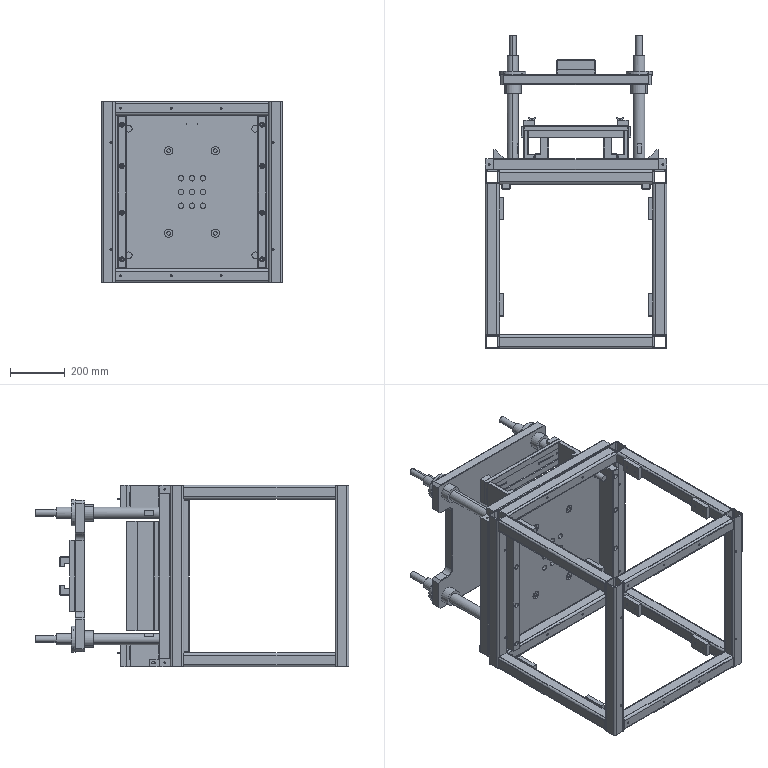Assembly | SolidWorks | mm | 35 component files | 54 solids | 2222 faces | box 660 x 1141 x 660 mm | volume 47833249 mm3 | cylinder 1006 | plane 864 | cone 344 | spline 8 | commonest cylinder face diameters 8.5 x176 5 x112 7 x100 6.8 x96 16 x48 8 x48 11 x48 10.5 x32
Bill of materials:
CHOB6-25 | 4 |  | Wing-head screw-like part: a plain cylindrical shank with a chamfered end, a short collar, a tapered conical hub, and two flat, angled wings sticking out on opposite sides of the hub.
DieBasePlate | 1 |  | Thin square flat plate with no visible holes or other features.
DieShim | 2 |  | Straight L-section (angle) bar with two groups of four small through-holes in a line along one leg.
GuidePlate | 2 |  | Long rectangular plate with a wide, shallow channel running its full length on one face, a hole near each corner, and two rows of small holes along the middle line toward each end.
GuidePlate1 | 4 |  | Rectangular block with a single obround (slotted) through-hole across its broad face.
GuideSupport | 4 |  | Short L-section bracket block with two round through-holes in one leg.
JJ01 | 1 |  | Open cube-shaped frame made of square hollow-section members. Four vertical corner posts are joined by four horizontal rails at the top and four at the bottom, leaving all six faces open. Small plates or tabs sit on the inner faces of the rails near the corners.
LowerReinforcement(2) | 2 |  | Narrow rectangular bar with four round through-holes along its length and two shallow cross grooves on one face near the ends.
Plate1 | 1 |  | Large, roughly square plate with stepped corner notches, a central 3x3 grid of holes, four larger holes near the corners, and many small holes and hole clusters spread across the face. Two opposite edges have a reduced-thickness step.
TriangularBracket | 2 |  | Right-angle corner block: a prism with two perpendicular outer faces, an angled (cut-off) face between them, and an obround through-slot in each perpendicular face.
UpperDieConnectingPlate1 | 1 |  | Rectangular plate with six very small holes in two rows of three, and small chamfers on the edges.
UpperDieShankSeat | 2 |  | Straight bar with an L-shaped (rabbeted) cross-section and three evenly spaced round through-holes on one long side face.
UpperDieSlidingPlate | 1 |  | Flat H-shaped plate: a rectangle with deep rectangular notches with rounded inner corners cut into two opposite sides, a round through-hole in each of the four corner lobes, and chamfered outer corners.
C-LHFR40LinearBearing | 4 |  | Flanged cylindrical bushing/sleeve: a hollow round tube with a through bore, joined at one end to a thin, larger-diameter circular flange that has four small through holes evenly spaced around a bolt circle.
UpperSupport | 4 |  | Solid stepped cylindrical shaft/pin: a long, larger-diameter central section with shorter, smaller-diameter coaxial sections at both ends, and a small local recess (possibly a keyway, slot or flat) on the central section near one end.
Mates:
1. coincident | UpperDieSlidingPlate-1 face at (-177.951, 623.269, 5) dir (0, 1, 0) | UpperDieConnectingPlate1-1 face at (-247.951, 623.269, 135) dir (0, -1, 0)
2. width | UpperDieConnectingPlate1-1 face at (-247.951, 643.269, -125) dir (0, 0, -1) | UpperDieConnectingPlate1-1 face at (-247.951, 643.269, 135) dir (0, 0, 1) | UpperDieSlidingPlate-1 face at (97.049, 623.269, -270) dir (0, 0, -1) | UpperDieSlidingPlate-1 face at (97.049, 623.269, 280) dir (0, 0, 1)
3. width | UpperDieConnectingPlate1-1 face at (-107.951, 643.269, 135) dir (1, 0, 0) | UpperDieConnectingPlate1-1 face at (-247.951, 643.269, 135) dir (-1, 0, 0) | UpperDieSlidingPlate-1 face at (-452.951, 623.269, 155) dir (-1, 0, 0) | UpperDieSlidingPlate-1 face at (97.049, 623.269, -270) dir (1, 0, 0)
4. coincident | UpperDieConnectingPlate1-1 face at (-247.951, 643.269, 135) dir (0, 1, 0) | UpperDieShankSeat-1 face at (-177.951, 643.269, 5) dir (0, -1, 0)
5. concentric | UpperDieConnectingPlate1-1 face at (-129.951, 643.269, 63) dir (0, 1, 0) r 4.25 | UpperDieShankSeat-1 face at (-129.951, 678.269, 63) dir (0, 1, 0) r 9
6. concentric | UpperDieConnectingPlate1-1 face at (-225.951, 643.269, 63) dir (0, 1, 0) r 4.25 | UpperDieShankSeat-1 face at (-225.951, 678.269, 63) dir (0, 1, 0) r 9
7. coincident | UpperDieConnectingPlate1-1 face at (-247.951, 643.269, 135) dir (0, 1, 0) | UpperDieShankSeat-2 face at (-177.951, 643.269, 5) dir (0, -1, 0)
8. concentric | UpperDieConnectingPlate1-1 face at (-225.951, 643.269, -53) dir (0, 1, 0) r 4.25 | UpperDieShankSeat-2 face at (-225.951, 678.269, -53) dir (0, 1, 0) r 9
9. concentric | UpperDieConnectingPlate1-1 face at (-129.951, 643.269, -53) dir (0, 1, 0) r 4.25 | UpperDieShankSeat-2 face at (-129.951, 678.269, -53) dir (0, 1, 0) r 9
10. coincident | DieShim-2 face at (-277.951, 397.323, 205) dir (0, 1, 0) | DieBasePlate-1 face at (-377.951, 397.323, 205) dir (0, -1, 0)
11. width | DieBasePlate-1 face at (-377.951, 437.323, 205) dir (0, 0, 1) | DieBasePlate-1 face at (-377.951, 437.323, -195) dir (0, 0, -1) | DieShim-1 face at (-77.951, 317.323, -195) dir (0, 0, -1) | DieShim-1 face at (-77.951, 317.323, 205) dir (0, 0, 1)
12. width | DieBasePlate-1 face at (22.049, 437.323, 205) dir (1, 0, 0) | DieBasePlate-1 face at (-377.951, 437.323, 205) dir (-1, 0, 0) | DieShim-2 face at (-307.951, 337.323, 205) dir (-1, 0, 0) | DieShim-1 face at (-47.951, 337.323, -195) dir (1, 0, 0)
13. coincident | DieBasePlate-1 face at (-377.951, 437.323, 205) dir (0, 1, 0) | GuidePlate-1 face at (-367.951, 437.323, -325) dir (0, 1, 0)
14. coincident | GuidePlate-1 face at (-367.951, 421.323, -325) dir (0, -1, 0) | GuideSupport-1 face at (-367.951, 421.323, -325) dir (0, 1, 0)
15. coincident | GuidePlate-1 face at (-367.951, 421.323, -325) dir (0, -1, 0) | GuideSupport-5 face at (12.049, 421.323, -225) dir (0, 1, 0)
16. coincident | GuidePlate-1 face at (-367.951, 437.323, -325) dir (0, 0, -1) | GuideSupport-5 face at (-3.951, 421.323, -325) dir (0, 0, -1)
17. concentric | GuidePlate-1 edge at (4.049, 436.323, -310) dir (0, 1, 0) r 2.75 | GuideSupport-5 edge at (4.049, 421.323, -310) dir (0, 1, 0) r 2.1
18. coincident | GuidePlate-1 face at (-367.951, 437.323, -325) dir (0, 0, -1) | GuideSupport-1 face at (-351.951, 421.323, -325) dir (0, 0, -1)
19. concentric | GuidePlate-1 edge at (-359.951, 437.323, -310) dir (0, -1, 0) r 3.75 | GuideSupport-1 edge at (-359.951, 421.323, -310) dir (0, 1, 0) r 2.1
20. coincident | GuidePlate-1 face at (-367.951, 437.323, -325) dir (0, 1, 0) | GuidePlate1-1 face at (-27.951, 437.323, -225) dir (0, -1, 0)
21. distance | GuidePlate1-1 face at (12.049, 437.323, -225) dir (1, 0, 0) | GuidePlate-1 face at (12.049, 437.323, -325) dir (1, 0, 0)
22. coincident | GuidePlate-1 face at (-367.951, 437.323, -325) dir (0, 0, -1) | GuidePlate1-1 face at (-27.951, 437.323, -325) dir (0, 0, -1)
23. coincident | GuidePlate1-1 face at (-27.951, 457.323, -225) dir (0, 1, 0) | CHOB6-25-1 face at (-22.201, 457.323, -275) dir (0, -1, 0)
24. concentric | GuidePlate1-1 face at (-17.951, 437.323, -275) dir (0, 1, 0) r 3.5 | CHOB6-25-1 face at (-17.951, 451.979, -275) dir (0, 1, 0) r 3
25. coincident | LowerReinforcement(2)-1 face at (92.049, 207.323, 280) dir (0, 0, 1) | LowerReinforcement(2)-2 face at (-417.951, 207.323, 280) dir (0, 0, 1)
26. coincident | LowerReinforcement(2)-1 face at (92.049, 207.323, -270) dir (0, -1, 0) | LowerReinforcement(2)-2 face at (-417.951, 207.323, -270) dir (0, -1, 0)
27. coincident | Plate1-2 face at (152.049, 317.323, 335) dir (0, 1, 0) | DieShim-1 face at (-56.625, 317.323, -195) dir (0, -1, 0)
28. distance | DieShim-1 face at (-27.951, 317.323, -195) dir (1, 0, 0) | Plate1-2 face at (152.049, 317.323, 335) dir (1, 0, 0)
29. width | GuidePlate-1 face at (12.049, 437.323, -325) dir (1, 0, 0) | GuidePlate-1 face at (-367.951, 437.323, -325) dir (-1, 0, 0) | Plate1-2 face at (-507.951, 317.323, 335) dir (-1, 0, 0) | Plate1-2 face at (152.049, 317.323, 335) dir (1, 0, 0)
30. coincident | Plate1-2 face at (152.049, 317.323, -325) dir (0, 0, -1) | GuidePlate-1 face at (-367.951, 437.323, -325) dir (0, 0, -1)
31. coincident | Plate1-2 face at (152.049, 277.323, 335) dir (0, -1, 0) | LowerReinforcement(2)-1 face at (92.049, 277.323, -270) dir (0, 1, 0)
32. distance | LowerReinforcement(2)-1 face at (92.049, 207.323, 280) dir (0, 0, 1) | Plate1-2 face at (152.049, 317.323, 335) dir (0, 0, 1)
33. distance | LowerReinforcement(2)-1 face at (92.049, 207.323, -270) dir (1, 0, 0) | Plate1-2 face at (152.049, 317.323, 335) dir (1, 0, 0)
34. distance | LowerReinforcement(2)-2 face at (-447.951, 207.323, -270) dir (-1, 0, 0) | Plate1-2 face at (-507.951, 317.323, 335) dir (-1, 0, 0)
35. coincident | Plate1-2 face at (152.049, 317.323, 335) dir (0, 1, 0) | TriangularBracket-5 face at (122.049, 317.323, -325) dir (0, -1, 0)
36. coincident | Plate1-2 face at (152.049, 317.323, -325) dir (0, 0, -1) | TriangularBracket-5 face at (122.049, 352.323, -325) dir (0, 0, -1)
37. coincident | Plate1-2 face at (152.049, 317.323, 335) dir (0, 1, 0) | TriangularBracket-6 face at (-477.951, 317.323, -297) dir (0, -1, 0)
38. width | DieBasePlate-1 face at (-377.951, 437.323, 205) dir (0, 0, 1) | DieBasePlate-1 face at (-377.951, 437.323, -195) dir (0, 0, -1) | Plate1-2 face at (152.049, 317.323, -325) dir (0, 0, -1) | Plate1-2 face at (152.049, 317.323, 335) dir (0, 0, 1)
39. concentric | UpperDieSlidingPlate-1 face at (52.049, 588.269, 235) dir (0, 1, 0) r 30 | UpperGuidePostAssembly-4/C-LHFR40LinearBearing-1 face at (52.049, 545.374, 235) dir (0, -1, 0) r 30
40. coincident | Plate1-2 face at (152.049, 317.323, 335) dir (0, 1, 0) | UpperGuidePostAssembly-4/UpperSupport-1 face at (52.693, 317.323, 246.983) dir (0, -1, 0)
41. width | UpperDieSlidingPlate-1 face at (97.049, 623.269, 155) dir (1, 0, 0) | UpperDieSlidingPlate-1 face at (-452.951, 623.269, 155) dir (-1, 0, 0) | Plate1-2 face at (-507.951, 317.323, 335) dir (-1, 0, 0) | Plate1-2 face at (152.049, 317.323, 335) dir (1, 0, 0)
42. width | UpperDieSlidingPlate-1 face at (97.049, 623.269, 280) dir (0, 0, 1) | UpperDieSlidingPlate-1 face at (97.049, 623.269, -270) dir (0, 0, -1) | Plate1-2 face at (152.049, 317.323, 335) dir (0, 0, 1) | Plate1-2 face at (152.049, 317.323, -325) dir (0, 0, -1)
43. concentric | UpperDieSlidingPlate-1 face at (-407.951, 588.269, 235) dir (0, 1, 0) r 30 | UpperGuidePostAssembly-2/C-LHFR40LinearBearing-1 face at (-407.951, 545.374, 235) dir (0, -1, 0) r 30
44. concentric | UpperDieSlidingPlate-1 face at (-407.951, 588.269, -225) dir (0, 1, 0) r 30 | UpperGuidePostAssembly-1/C-LHFR40LinearBearing-1 face at (-407.951, 545.374, -225) dir (0, -1, 0) r 30
45. concentric | UpperDieSlidingPlate-1 face at (52.049, 588.269, -225) dir (0, 1, 0) r 30 | UpperGuidePostAssembly-3/C-LHFR40LinearBearing-1 face at (52.049, 545.374, -225) dir (0, -1, 0) r 30
46. coincident | UpperDieSlidingPlate-1 face at (-177.951, 623.269, 5) dir (0, 1, 0) | UpperGuidePostAssembly-3/C-LHFR40LinearBearing-1 face at (18.108, 623.269, -191.059) dir (0, -1, 0)
47. coincident | UpperGuidePostAssembly-3/UpperSupport-1 face at (72.049, 692.323, -225) dir (0, 1, 0) | UpperGuidePostAssembly-4/UpperSupport-1 face at (53.123, 692.323, 254.971) dir (0, 1, 0)
48. coincident | UpperGuidePostAssembly-2/UpperSupport-1 face at (-387.951, 692.323, 235) dir (0, 1, 0) | UpperGuidePostAssembly-4/UpperSupport-1 face at (53.123, 692.323, 254.971) dir (0, 1, 0)
49. coincident | UpperGuidePostAssembly-1/UpperSupport-1 face at (-419.494, 692.323, -208.668) dir (0, 1, 0) | UpperGuidePostAssembly-2/UpperSupport-1 face at (-387.951, 692.323, 235) dir (0, 1, 0)
50. coincident | UpperGuidePostAssembly-3/C-LHFR40LinearBearing-1 face at (37.907, 636.269, -210.858) dir (0, 1, 0) | UpperGuidePostAssembly-4/C-LHFR40LinearBearing-1 face at (37.907, 636.269, 249.142) dir (0, 1, 0)
51. coincident | UpperGuidePostAssembly-2/C-LHFR40LinearBearing-1 face at (-393.809, 636.269, 249.142) dir (0, 1, 0) | UpperGuidePostAssembly-4/C-LHFR40LinearBearing-1 face at (37.907, 636.269, 249.142) dir (0, 1, 0)
52. coincident | UpperGuidePostAssembly-1/C-LHFR40LinearBearing-1 face at (-422.093, 636.269, -210.858) dir (0, 1, 0) | UpperGuidePostAssembly-2/C-LHFR40LinearBearing-1 face at (-393.809, 636.269, 249.142) dir (0, 1, 0)
53. concentric | UpperDieSlidingPlate-1 face at (79.626, 623.269, -252.577) dir (0, 1, 0) r 3.4 | UpperGuidePostAssembly-3/C-LHFR40LinearBearing-1 face at (79.626, 636.269, -252.577) dir (0, 1, 0) r 4.5
54. concentric | UpperDieSlidingPlate-1 face at (-380.374, 623.269, -252.577) dir (0, 1, 0) r 3.4 | UpperGuidePostAssembly-1/C-LHFR40LinearBearing-1 face at (-380.374, 636.269, -252.577) dir (0, 1, 0) r 4.5
55. concentric | UpperDieSlidingPlate-1 face at (-435.528, 623.269, 262.577) dir (0, 1, 0) r 3.4 | UpperGuidePostAssembly-2/C-LHFR40LinearBearing-1 face at (-435.528, 636.269, 262.577) dir (0, 1, 0) r 4.5
56. concentric | UpperDieSlidingPlate-1 face at (79.626, 623.269, 262.577) dir (0, 1, 0) r 3.4 | UpperGuidePostAssembly-4/C-LHFR40LinearBearing-1 face at (79.626, 636.269, 262.577) dir (0, 1, 0) r 4.5
57. coincident | JJ01-1 face at (127.049, 235.323, -325) dir (0, 0, -1) | TriangularBracket-6 face at (-477.951, 352.323, -325) dir (0, 0, -1)
58. coincident | JJ01-1 face at (-482.951, 277.323, 293) dir (0, 1, 0) | Plate1-2 face at (152.049, 277.323, 335) dir (0, -1, 0)
59. coincident | JJ01-1 face at (152.049, 235.323, -300) dir (1, 0, 0) | Plate1-2 face at (152.049, 317.323, 335) dir (1, 0, 0)
60. width | JJ01-1 face at (-482.951, 235.323, 335) dir (0, 0, 1) | JJ01-1 face at (127.049, 235.323, -325) dir (0, 0, -1) | Plate1-2 face at (152.049, 317.323, -325) dir (0, 0, -1) | Plate1-2 face at (152.049, 317.323, 335) dir (0, 0, 1)
61. concentric | UpperSupport-1 face at (-14.085, 6.786, 80.197) dir (0, 0, -1) r 20 | C-LHFR40LinearBearing-1 face at (-14.085, 6.786, 303.145) dir (0, 0, 1) r 30
62. distance | C-LHFR40LinearBearing-1 face at (1.97, 18.712, 212.25) dir (0, 0, -1) | UpperSupport-1 face at (5.915, 6.786, 156.197) dir (0, 0, -1)